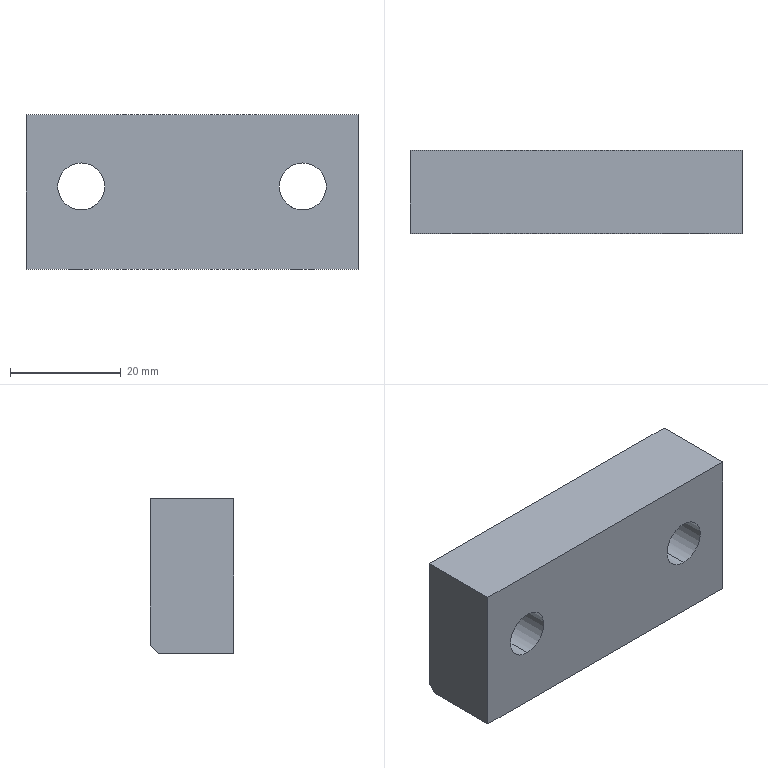Component | SolidWorks | Q1-A12-S21-Q4E.SLDASQ-5_Q1-A12-S21-Q1E-02A-1 | 1 solid | 15 faces | box 60 x 15 x 28 mm | volume 23129 mm3 | cylinder 8 | plane 7 | commonest cylinder face diameters 8.5 x4 4.2 x4 | material Q235-Steel
build123d program:
from build123d import *

# Parameters (mm, degrees)
SKETCH1_W                  = 60
SKETCH1_H                  = 28
BOSS_EXTRUDE1_DEPTH        = 15
M5X0_8_TAPPED_HOLE1_D      = 4.2
M5X0_8_TAPPED_HOLE1_DEPTH  = 12.4
M5X0_8_TAPPED_HOLE1_TIP    = 1.262
F_8_5_8_5_DIAMETER_HOLE1_D = 8.5
CHAMFER1_SIZE              = 1.5


with BuildPart() as part:
    # Sketch1 → Boss-Extrude1 (new body)
    with BuildSketch(Plane(origin=(0, 0, 0), x_dir=(1, 0, 0), z_dir=(0, 1, 0))):
        Rectangle(SKETCH1_W, SKETCH1_H)
    extrude(amount=BOSS_EXTRUDE1_DEPTH)

    # M5x0.8 Tapped Hole1
    with Locations(Plane(origin=(0, 0, -14), x_dir=(-1, 0, 0), z_dir=(0, 0, -1))):
        with Locations((20, 7.5), (-20, 7.5)):
            Hole(M5X0_8_TAPPED_HOLE1_D / 2, depth=M5X0_8_TAPPED_HOLE1_DEPTH)
            with Locations((0, 0, -(M5X0_8_TAPPED_HOLE1_DEPTH + M5X0_8_TAPPED_HOLE1_TIP / 2))):  # 118° drill point
                Cone(0, M5X0_8_TAPPED_HOLE1_D / 2, M5X0_8_TAPPED_HOLE1_TIP, mode=Mode.SUBTRACT)

    # 8.5 _8.5_ Diameter Hole1 (through all)
    with Locations(Plane(origin=(0, 15, 0), x_dir=(1, 0, 0), z_dir=(0, 1, 0))):
        with Locations((-20, -1), (20, -1)):
            Hole(F_8_5_8_5_DIAMETER_HOLE1_D / 2)

    # Chamfer1
    chamfer1_edges = [part.edges().sort_by_distance(p)[0] for p in [
        (0, 15, -14),
    ]]
    chamfer(chamfer1_edges, length=CHAMFER1_SIZE)


solid = part.part

# Placed as in the assembly
solid = solid.moved(Location((1198.5, -55, 174), (0, 0, 0)))
STEP:
#1=COLOUR_RGB('',0.7922,0.8196,0.9333);
#2=FILL_AREA_STYLE_COLOUR('',#1);
#3=FILL_AREA_STYLE('',(#2));
#4=SURFACE_STYLE_FILL_AREA(#3);
#5=SURFACE_SIDE_STYLE('',(#4));
#6=SURFACE_STYLE_USAGE(.BOTH.,#5);
#7=PRESENTATION_STYLE_ASSIGNMENT((#6));
#8=CARTESIAN_POINT('',(46.398,-2.165,6.722));
#9=VERTEX_POINT('',#8);
#10=CARTESIAN_POINT('',(46.398,-2.165,7.057));
#11=VERTEX_POINT('',#10);
#12=CARTESIAN_POINT('',(46.398,-2.165,6.89));
#13=DIRECTION('',(0.,1.,0.));
#14=DIRECTION('',(0.,0.,1.));
#15=AXIS2_PLACEMENT_3D('',#12,#13,#14);
#16=CIRCLE('',#15,0.1673);
#17=EDGE_CURVE('',#9,#11,#16,.T.);
#18=ORIENTED_EDGE('',*,*,#17,.F.);
#19=CARTESIAN_POINT('',(46.398,-1.953,6.722));
#20=VERTEX_POINT('',#19);
#21=CARTESIAN_POINT('',(46.398,-1.575,6.722));
#22=DIRECTION('',(0.,1.,0.));
#23=VECTOR('',#22,39.37);
#24=LINE('',#21,#23);
#25=EDGE_CURVE('',#9,#20,#24,.T.);
#26=ORIENTED_EDGE('',*,*,#25,.T.);
#27=CARTESIAN_POINT('',(46.315,-1.87,6.744));
#28=VERTEX_POINT('',#27);
#29=CARTESIAN_POINT('',(46.315,-1.87,6.744));
#30=CARTESIAN_POINT('',(46.315,-1.876,6.744));
#31=CARTESIAN_POINT('',(46.316,-1.881,6.744));
#32=CARTESIAN_POINT('',(46.318,-1.892,6.743));
#33=CARTESIAN_POINT('',(46.319,-1.897,6.742));
#34=CARTESIAN_POINT('',(46.326,-1.912,6.739));
#35=CARTESIAN_POINT('',(46.332,-1.921,6.736));
#36=CARTESIAN_POINT('',(46.347,-1.936,6.73));
#37=CARTESIAN_POINT('',(46.356,-1.942,6.727));
#38=CARTESIAN_POINT('',(46.371,-1.948,6.725));
#39=CARTESIAN_POINT('',(46.376,-1.95,6.724));
#40=CARTESIAN_POINT('',(46.387,-1.952,6.723));
#41=CARTESIAN_POINT('',(46.392,-1.953,6.722));
#42=CARTESIAN_POINT('',(46.398,-1.953,6.722));
#43=B_SPLINE_CURVE_WITH_KNOTS('',3,(#29,#30,#31,#32,#33,#34,#35,#36,#37,#38,#39,#40,#41,#42),.UNSPECIFIED.,.F.,.F.,(4,2,2,2,2,2,4),(0.,0.0004174,0.0008349,0.00167,0.002505,0.002922,0.003339),.UNSPECIFIED.);
#44=EDGE_CURVE('',#28,#20,#43,.T.);
#45=ORIENTED_EDGE('',*,*,#44,.F.);
#46=CARTESIAN_POINT('',(46.398,-1.787,6.722));
#47=VERTEX_POINT('',#46);
#48=CARTESIAN_POINT('',(46.398,-1.787,6.722));
#49=CARTESIAN_POINT('',(46.392,-1.787,6.722));
#50=CARTESIAN_POINT('',(46.387,-1.788,6.723));
#51=CARTESIAN_POINT('',(46.376,-1.79,6.724));
#52=CARTESIAN_POINT('',(46.371,-1.792,6.725));
#53=CARTESIAN_POINT('',(46.356,-1.798,6.727));
#54=CARTESIAN_POINT('',(46.347,-1.804,6.73));
#55=CARTESIAN_POINT('',(46.335,-1.815,6.734));
#56=CARTESIAN_POINT('',(46.332,-1.82,6.736));
#57=CARTESIAN_POINT('',(46.326,-1.828,6.738));
#58=CARTESIAN_POINT('',(46.323,-1.833,6.74));
#59=CARTESIAN_POINT('',(46.319,-1.843,6.742));
#60=CARTESIAN_POINT('',(46.318,-1.848,6.743));
#61=CARTESIAN_POINT('',(46.316,-1.859,6.744));
#62=CARTESIAN_POINT('',(46.315,-1.865,6.744));
#63=CARTESIAN_POINT('',(46.315,-1.87,6.744));
#64=B_SPLINE_CURVE_WITH_KNOTS('',3,(#48,#49,#50,#51,#52,#53,#54,#55,#56,#57,#58,#59,#60,#61,#62,#63),.UNSPECIFIED.,.F.,.F.,(4,2,2,2,2,2,2,4),(0.01001,0.01043,0.01084,0.01168,0.01209,0.01251,0.01292,0.01334),.UNSPECIFIED.);
#65=EDGE_CURVE('',#47,#28,#64,.T.);
#66=ORIENTED_EDGE('',*,*,#65,.F.);
#67=CARTESIAN_POINT('',(46.398,-1.575,6.722));
#68=VERTEX_POINT('',#67);
#69=CARTESIAN_POINT('',(46.398,-1.575,6.722));
#70=DIRECTION('',(0.,1.,0.));
#71=VECTOR('',#70,39.37);
#72=LINE('',#69,#71);
#73=EDGE_CURVE('',#47,#68,#72,.T.);
#74=ORIENTED_EDGE('',*,*,#73,.T.);
#75=CARTESIAN_POINT('',(46.398,-1.575,7.057));
#76=VERTEX_POINT('',#75);
#77=CARTESIAN_POINT('',(46.398,-1.575,6.89));
#78=DIRECTION('',(0.,1.,0.));
#79=DIRECTION('',(0.,0.,1.));
#80=AXIS2_PLACEMENT_3D('',#77,#78,#79);
#81=CIRCLE('',#80,0.1673);
#82=EDGE_CURVE('',#68,#76,#81,.T.);
#83=ORIENTED_EDGE('',*,*,#82,.T.);
#84=CARTESIAN_POINT('',(46.398,-1.575,7.057));
#85=DIRECTION('',(0.,1.,0.));
#86=VECTOR('',#85,39.37);
#87=LINE('',#84,#86);
#88=EDGE_CURVE('',#11,#76,#87,.T.);
#89=ORIENTED_EDGE('',*,*,#88,.F.);
#90=EDGE_LOOP('',(#18,#26,#45,#66,#74,#83,#89));
#91=FACE_OUTER_BOUND('',#90,.T.);
#92=CARTESIAN_POINT('',(46.398,-1.575,6.89));
#93=DIRECTION('',(0.,1.,0.));
#94=DIRECTION('',(0.,0.,1.));
#95=AXIS2_PLACEMENT_3D('',#92,#93,#94);
#96=CYLINDRICAL_SURFACE('',#95,0.1673);
#97=ADVANCED_FACE('',(#91),#96,.F.);
#98=CARTESIAN_POINT('',(47.972,-2.165,6.722));
#99=VERTEX_POINT('',#98);
#100=CARTESIAN_POINT('',(47.972,-2.165,7.057));
#101=VERTEX_POINT('',#100);
#102=CARTESIAN_POINT('',(47.972,-2.165,6.89));
#103=DIRECTION('',(0.,1.,0.));
#104=DIRECTION('',(0.,0.,1.));
#105=AXIS2_PLACEMENT_3D('',#102,#103,#104);
#106=CIRCLE('',#105,0.1673);
#107=EDGE_CURVE('',#99,#101,#106,.T.);
#108=ORIENTED_EDGE('',*,*,#107,.F.);
#109=CARTESIAN_POINT('',(47.972,-1.953,6.722));
#110=VERTEX_POINT('',#109);
#111=CARTESIAN_POINT('',(47.972,-1.575,6.722));
#112=DIRECTION('',(0.,1.,0.));
#113=VECTOR('',#112,39.37);
#114=LINE('',#111,#113);
#115=EDGE_CURVE('',#99,#110,#114,.T.);
#116=ORIENTED_EDGE('',*,*,#115,.T.);
#117=CARTESIAN_POINT('',(47.89,-1.87,6.744));
#118=VERTEX_POINT('',#117);
#119=CARTESIAN_POINT('',(47.89,-1.87,6.744));
#120=CARTESIAN_POINT('',(47.89,-1.876,6.744));
#121=CARTESIAN_POINT('',(47.89,-1.881,6.744));
#122=CARTESIAN_POINT('',(47.892,-1.892,6.743));
#123=CARTESIAN_POINT('',(47.894,-1.897,6.742));
#124=CARTESIAN_POINT('',(47.9,-1.912,6.739));
#125=CARTESIAN_POINT('',(47.906,-1.921,6.736));
#126=CARTESIAN_POINT('',(47.921,-1.936,6.73));
#127=CARTESIAN_POINT('',(47.931,-1.942,6.727));
#128=CARTESIAN_POINT('',(47.945,-1.948,6.725));
#129=CARTESIAN_POINT('',(47.951,-1.95,6.724));
#130=CARTESIAN_POINT('',(47.961,-1.952,6.723));
#131=CARTESIAN_POINT('',(47.967,-1.953,6.722));
#132=CARTESIAN_POINT('',(47.972,-1.953,6.722));
#133=B_SPLINE_CURVE_WITH_KNOTS('',3,(#119,#120,#121,#122,#123,#124,#125,#126,#127,#128,#129,#130,#131,#132),.UNSPECIFIED.,.F.,.F.,(4,2,2,2,2,2,4),(0.,0.0004174,0.0008349,0.00167,0.002505,0.002922,0.003339),.UNSPECIFIED.);
#134=EDGE_CURVE('',#118,#110,#133,.T.);
#135=ORIENTED_EDGE('',*,*,#134,.F.);
#136=CARTESIAN_POINT('',(47.972,-1.787,6.722));
#137=VERTEX_POINT('',#136);
#138=CARTESIAN_POINT('',(47.972,-1.787,6.722));
#139=CARTESIAN_POINT('',(47.967,-1.787,6.722));
#140=CARTESIAN_POINT('',(47.961,-1.788,6.723));
#141=CARTESIAN_POINT('',(47.951,-1.79,6.724));
#142=CARTESIAN_POINT('',(47.945,-1.792,6.725));
#143=CARTESIAN_POINT('',(47.93,-1.798,6.727));
#144=CARTESIAN_POINT('',(47.921,-1.804,6.73));
#145=CARTESIAN_POINT('',(47.91,-1.815,6.734));
#146=CARTESIAN_POINT('',(47.907,-1.82,6.736));
#147=CARTESIAN_POINT('',(47.901,-1.828,6.738));
#148=CARTESIAN_POINT('',(47.898,-1.833,6.74));
#149=CARTESIAN_POINT('',(47.894,-1.843,6.742));
#150=CARTESIAN_POINT('',(47.893,-1.848,6.743));
#151=CARTESIAN_POINT('',(47.89,-1.859,6.744));
#152=CARTESIAN_POINT('',(47.89,-1.865,6.744));
#153=CARTESIAN_POINT('',(47.89,-1.87,6.744));
#154=B_SPLINE_CURVE_WITH_KNOTS('',3,(#138,#139,#140,#141,#142,#143,#144,#145,#146,#147,#148,#149,#150,#151,#152,#153),.UNSPECIFIED.,.F.,.F.,(4,2,2,2,2,2,2,4),(0.01001,0.01043,0.01084,0.01168,0.01209,0.01251,0.01292,0.01334),.UNSPECIFIED.);
#155=EDGE_CURVE('',#137,#118,#154,.T.);
#156=ORIENTED_EDGE('',*,*,#155,.F.);
#157=CARTESIAN_POINT('',(47.972,-1.575,6.722));
#158=VERTEX_POINT('',#157);
#159=CARTESIAN_POINT('',(47.972,-1.575,6.722));
#160=DIRECTION('',(0.,1.,0.));
#161=VECTOR('',#160,39.37);
#162=LINE('',#159,#161);
#163=EDGE_CURVE('',#137,#158,#162,.T.);
#164=ORIENTED_EDGE('',*,*,#163,.T.);
#165=CARTESIAN_POINT('',(47.972,-1.575,7.057));
#166=VERTEX_POINT('',#165);
#167=CARTESIAN_POINT('',(47.972,-1.575,6.89));
#168=DIRECTION('',(0.,1.,0.));
#169=DIRECTION('',(0.,0.,1.));
#170=AXIS2_PLACEMENT_3D('',#167,#168,#169);
#171=CIRCLE('',#170,0.1673);
#172=EDGE_CURVE('',#158,#166,#171,.T.);
#173=ORIENTED_EDGE('',*,*,#172,.T.);
#174=CARTESIAN_POINT('',(47.972,-1.575,7.057));
#175=DIRECTION('',(0.,1.,0.));
#176=VECTOR('',#175,39.37);
#177=LINE('',#174,#176);
#178=EDGE_CURVE('',#101,#166,#177,.T.);
#179=ORIENTED_EDGE('',*,*,#178,.F.);
#180=EDGE_LOOP('',(#108,#116,#135,#156,#164,#173,#179));
#181=FACE_OUTER_BOUND('',#180,.T.);
#182=CARTESIAN_POINT('',(47.972,-1.575,6.89));
#183=DIRECTION('',(0.,1.,0.));
#184=DIRECTION('',(0.,0.,1.));
#185=AXIS2_PLACEMENT_3D('',#182,#183,#184);
#186=CYLINDRICAL_SURFACE('',#185,0.1673);
#187=ADVANCED_FACE('',(#181),#186,.F.);
#188=ORIENTED_EDGE('',*,*,#44,.T.);
#189=CARTESIAN_POINT('',(46.48,-1.87,6.744));
#190=VERTEX_POINT('',#189);
#191=CARTESIAN_POINT('',(46.398,-1.953,6.722));
#192=CARTESIAN_POINT('',(46.403,-1.953,6.722));
#193=CARTESIAN_POINT('',(46.409,-1.952,6.723));
#194=CARTESIAN_POINT('',(46.419,-1.95,6.724));
#195=CARTESIAN_POINT('',(46.425,-1.948,6.725));
#196=CARTESIAN_POINT('',(46.435,-1.944,6.727));
#197=CARTESIAN_POINT('',(46.439,-1.942,6.728));
#198=CARTESIAN_POINT('',(46.448,-1.936,6.73));
#199=CARTESIAN_POINT('',(46.452,-1.932,6.732));
#200=CARTESIAN_POINT('',(46.464,-1.921,6.736));
#201=CARTESIAN_POINT('',(46.47,-1.912,6.739));
#202=CARTESIAN_POINT('',(46.476,-1.897,6.742));
#203=CARTESIAN_POINT('',(46.478,-1.892,6.743));
#204=CARTESIAN_POINT('',(46.48,-1.881,6.744));
#205=CARTESIAN_POINT('',(46.48,-1.876,6.744));
#206=CARTESIAN_POINT('',(46.48,-1.87,6.744));
#207=B_SPLINE_CURVE_WITH_KNOTS('',3,(#191,#192,#193,#194,#195,#196,#197,#198,#199,#200,#201,#202,#203,#204,#205,#206),.UNSPECIFIED.,.F.,.F.,(4,2,2,2,2,2,2,4),(0.003339,0.003757,0.004174,0.004591,0.005008,0.005842,0.006259,0.006676),.UNSPECIFIED.);
#208=EDGE_CURVE('',#20,#190,#207,.T.);
#209=ORIENTED_EDGE('',*,*,#208,.T.);
#210=CARTESIAN_POINT('',(46.48,-1.87,6.299));
#211=VERTEX_POINT('',#210);
#212=CARTESIAN_POINT('',(46.48,-1.87,6.299));
#213=DIRECTION('',(0.,0.,-1.));
#214=VECTOR('',#213,39.37);
#215=LINE('',#212,#214);
#216=EDGE_CURVE('',#190,#211,#215,.T.);
#217=ORIENTED_EDGE('',*,*,#216,.T.);
#218=CARTESIAN_POINT('',(46.315,-1.87,6.299));
#219=VERTEX_POINT('',#218);
#220=CARTESIAN_POINT('',(46.398,-1.87,6.299));
#221=DIRECTION('',(0.,0.,-1.));
#222=DIRECTION('',(-1.,0.,0.));
#223=AXIS2_PLACEMENT_3D('',#220,#221,#222);
#224=CIRCLE('',#223,0.08268);
#225=EDGE_CURVE('',#211,#219,#224,.T.);
#226=ORIENTED_EDGE('',*,*,#225,.T.);
#227=CARTESIAN_POINT('',(46.315,-1.87,6.299));
#228=DIRECTION('',(0.,0.,-1.));
#229=VECTOR('',#228,39.37);
#230=LINE('',#227,#229);
#231=EDGE_CURVE('',#28,#219,#230,.T.);
#232=ORIENTED_EDGE('',*,*,#231,.F.);
#233=EDGE_LOOP('',(#188,#209,#217,#226,#232));
#234=FACE_OUTER_BOUND('',#233,.T.);
#235=CARTESIAN_POINT('',(46.398,-1.87,6.299));
#236=DIRECTION('',(0.,0.,-1.));
#237=DIRECTION('',(-1.,0.,0.));
#238=AXIS2_PLACEMENT_3D('',#235,#236,#237);
#239=CYLINDRICAL_SURFACE('',#238,0.08268);
#240=ADVANCED_FACE('',(#234),#239,.F.);
#241=ORIENTED_EDGE('',*,*,#134,.T.);
#242=CARTESIAN_POINT('',(48.055,-1.87,6.744));
#243=VERTEX_POINT('',#242);
#244=CARTESIAN_POINT('',(47.972,-1.953,6.722));
#245=CARTESIAN_POINT('',(47.978,-1.953,6.722));
#246=CARTESIAN_POINT('',(47.984,-1.952,6.723));
#247=CARTESIAN_POINT('',(47.994,-1.95,6.724));
#248=CARTESIAN_POINT('',(47.999,-1.948,6.725));
#249=CARTESIAN_POINT('',(48.009,-1.944,6.727));
#250=CARTESIAN_POINT('',(48.014,-1.942,6.728));
#251=CARTESIAN_POINT('',(48.023,-1.936,6.73));
#252=CARTESIAN_POINT('',(48.027,-1.932,6.732));
#253=CARTESIAN_POINT('',(48.039,-1.921,6.736));
#254=CARTESIAN_POINT('',(48.045,-1.912,6.739));
#255=CARTESIAN_POINT('',(48.051,-1.897,6.742));
#256=CARTESIAN_POINT('',(48.052,-1.892,6.743));
#257=CARTESIAN_POINT('',(48.055,-1.881,6.744));
#258=CARTESIAN_POINT('',(48.055,-1.876,6.744));
#259=CARTESIAN_POINT('',(48.055,-1.87,6.744));
#260=B_SPLINE_CURVE_WITH_KNOTS('',3,(#244,#245,#246,#247,#248,#249,#250,#251,#252,#253,#254,#255,#256,#257,#258,#259),.UNSPECIFIED.,.F.,.F.,(4,2,2,2,2,2,2,4),(0.003339,0.003757,0.004174,0.004591,0.005008,0.005842,0.006259,0.006676),.UNSPECIFIED.);
#261=EDGE_CURVE('',#110,#243,#260,.T.);
#262=ORIENTED_EDGE('',*,*,#261,.T.);
#263=CARTESIAN_POINT('',(48.055,-1.87,6.299));
#264=VERTEX_POINT('',#263);
#265=CARTESIAN_POINT('',(48.055,-1.87,6.299));
#266=DIRECTION('',(0.,0.,-1.));
#267=VECTOR('',#266,39.37);
#268=LINE('',#265,#267);
#269=EDGE_CURVE('',#243,#264,#268,.T.);
#270=ORIENTED_EDGE('',*,*,#269,.T.);
#271=CARTESIAN_POINT('',(47.89,-1.87,6.299));
#272=VERTEX_POINT('',#271);
#273=CARTESIAN_POINT('',(47.972,-1.87,6.299));
#274=DIRECTION('',(0.,0.,-1.));
#275=DIRECTION('',(-1.,0.,0.));
#276=AXIS2_PLACEMENT_3D('',#273,#274,#275);
#277=CIRCLE('',#276,0.08268);
#278=EDGE_CURVE('',#264,#272,#277,.T.);
#279=ORIENTED_EDGE('',*,*,#278,.T.);
#280=CARTESIAN_POINT('',(47.89,-1.87,6.299));
#281=DIRECTION('',(0.,0.,-1.));
#282=VECTOR('',#281,39.37);
#283=LINE('',#280,#282);
#284=EDGE_CURVE('',#118,#272,#283,.T.);
#285=ORIENTED_EDGE('',*,*,#284,.F.);
#286=EDGE_LOOP('',(#241,#262,#270,#279,#285));
#287=FACE_OUTER_BOUND('',#286,.T.);
#288=CARTESIAN_POINT('',(47.972,-1.87,6.299));
#289=DIRECTION('',(0.,0.,-1.));
#290=DIRECTION('',(-1.,0.,0.));
#291=AXIS2_PLACEMENT_3D('',#288,#289,#290);
#292=CYLINDRICAL_SURFACE('',#291,0.08268);
#293=ADVANCED_FACE('',(#287),#292,.F.);
#294=CARTESIAN_POINT('',(48.366,-1.634,6.299));
#295=VERTEX_POINT('',#294);
#296=CARTESIAN_POINT('',(48.366,-2.165,6.299));
#297=VERTEX_POINT('',#296);
#298=CARTESIAN_POINT('',(48.366,-1.575,6.299));
#299=DIRECTION('',(0.,-1.,0.));
#300=VECTOR('',#299,39.37);
#301=LINE('',#298,#300);
#302=EDGE_CURVE('',#295,#297,#301,.T.);
#303=ORIENTED_EDGE('',*,*,#302,.F.);
#304=CARTESIAN_POINT('',(48.366,-1.575,6.358));
#305=VERTEX_POINT('',#304);
#306=CARTESIAN_POINT('',(48.366,-1.575,6.358));
#307=DIRECTION('',(0.,0.7071,0.7071));
#308=VECTOR('',#307,39.37);
#309=LINE('',#306,#308);
#310=EDGE_CURVE('',#295,#305,#309,.T.);
#311=ORIENTED_EDGE('',*,*,#310,.T.);
#312=CARTESIAN_POINT('',(48.366,-1.575,7.402));
#313=VERTEX_POINT('',#312);
#314=CARTESIAN_POINT('',(48.366,-1.575,7.402));
#315=DIRECTION('',(0.,0.,-1.));
#316=VECTOR('',#315,39.37);
#317=LINE('',#314,#316);
#318=EDGE_CURVE('',#313,#305,#317,.T.);
#319=ORIENTED_EDGE('',*,*,#318,.F.);
#320=CARTESIAN_POINT('',(48.366,-2.165,7.402));
#321=VERTEX_POINT('',#320);
#322=CARTESIAN_POINT('',(48.366,-1.575,7.402));
#323=DIRECTION('',(0.,-1.,0.));
#324=VECTOR('',#323,39.37);
#325=LINE('',#322,#324);
#326=EDGE_CURVE('',#313,#321,#325,.T.);
#327=ORIENTED_EDGE('',*,*,#326,.T.);
#328=CARTESIAN_POINT('',(48.366,-2.165,7.402));
#329=DIRECTION('',(0.,0.,-1.));
#330=VECTOR('',#329,39.37);
#331=LINE('',#328,#330);
#332=EDGE_CURVE('',#321,#297,#331,.T.);
#333=ORIENTED_EDGE('',*,*,#332,.T.);
#334=EDGE_LOOP('',(#303,#311,#319,#327,#333));
#335=FACE_OUTER_BOUND('',#334,.T.);
#336=CARTESIAN_POINT('',(48.366,-1.575,7.402));
#337=DIRECTION('',(-1.,0.,0.));
#338=DIRECTION('',(0.,0.,1.));
#339=AXIS2_PLACEMENT_3D('',#336,#337,#338);
#340=PLANE('',#339);
#341=ADVANCED_FACE('',(#335),#340,.F.);
#342=CARTESIAN_POINT('',(46.398,-1.87,6.299));
#343=DIRECTION('',(0.,0.,-1.));
#344=DIRECTION('',(-1.,0.,0.));
#345=AXIS2_PLACEMENT_3D('',#342,#343,#344);
#346=CIRCLE('',#345,0.08268);
#347=EDGE_CURVE('',#219,#211,#346,.T.);
#348=ORIENTED_EDGE('',*,*,#347,.F.);
#349=ORIENTED_EDGE('',*,*,#225,.F.);
#350=EDGE_LOOP('',(#348,#349));
#351=FACE_BOUND('',#350,.T.);
#352=CARTESIAN_POINT('',(47.972,-1.87,6.299));
#353=DIRECTION('',(0.,0.,-1.));
#354=DIRECTION('',(-1.,0.,0.));
#355=AXIS2_PLACEMENT_3D('',#352,#353,#354);
#356=CIRCLE('',#355,0.08268);
#357=EDGE_CURVE('',#272,#264,#356,.T.);
#358=ORIENTED_EDGE('',*,*,#357,.F.);
#359=ORIENTED_EDGE('',*,*,#278,.F.);
#360=EDGE_LOOP('',(#358,#359));
#361=FACE_BOUND('',#360,.T.);
#362=CARTESIAN_POINT('',(46.004,-1.634,6.299));
#363=VERTEX_POINT('',#362);
#364=CARTESIAN_POINT('',(46.004,-2.165,6.299));
#365=VERTEX_POINT('',#364);
#366=CARTESIAN_POINT('',(46.004,-1.575,6.299));
#367=DIRECTION('',(0.,-1.,0.));
#368=VECTOR('',#367,39.37);
#369=LINE('',#366,#368);
#370=EDGE_CURVE('',#363,#365,#369,.T.);
#371=ORIENTED_EDGE('',*,*,#370,.F.);
#372=CARTESIAN_POINT('',(46.004,-1.634,6.299));
#373=DIRECTION('',(1.,0.,0.));
#374=VECTOR('',#373,39.37);
#375=LINE('',#372,#374);
#376=EDGE_CURVE('',#363,#295,#375,.T.);
#377=ORIENTED_EDGE('',*,*,#376,.T.);
#378=ORIENTED_EDGE('',*,*,#302,.T.);
#379=CARTESIAN_POINT('',(46.004,-2.165,6.299));
#380=DIRECTION('',(-1.,0.,0.));
#381=VECTOR('',#380,39.37);
#382=LINE('',#379,#381);
#383=EDGE_CURVE('',#297,#365,#382,.T.);
#384=ORIENTED_EDGE('',*,*,#383,.T.);
#385=EDGE_LOOP('',(#371,#377,#378,#384));
#386=FACE_OUTER_BOUND('',#385,.T.);
#387=CARTESIAN_POINT('',(46.004,-1.575,6.299));
#388=DIRECTION('',(0.,0.,1.));
#389=DIRECTION('',(1.,0.,0.));
#390=AXIS2_PLACEMENT_3D('',#387,#388,#389);
#391=PLANE('',#390);
#392=ADVANCED_FACE('',(#351,#361,#386),#391,.F.);
#393=CARTESIAN_POINT('',(46.004,-1.575,6.358));
#394=VERTEX_POINT('',#393);
#395=CARTESIAN_POINT('',(46.004,-1.575,7.402));
#396=VERTEX_POINT('',#395);
#397=CARTESIAN_POINT('',(46.004,-1.575,7.402));
#398=DIRECTION('',(0.,0.,1.));
#399=VECTOR('',#398,39.37);
#400=LINE('',#397,#399);
#401=EDGE_CURVE('',#394,#396,#400,.T.);
#402=ORIENTED_EDGE('',*,*,#401,.F.);
#403=CARTESIAN_POINT('',(46.004,-1.575,6.358));
#404=DIRECTION('',(0.,-0.7071,-0.7071));
#405=VECTOR('',#404,39.37);
#406=LINE('',#403,#405);
#407=EDGE_CURVE('',#394,#363,#406,.T.);
#408=ORIENTED_EDGE('',*,*,#407,.T.);
#409=ORIENTED_EDGE('',*,*,#370,.T.);
#410=CARTESIAN_POINT('',(46.004,-2.165,7.402));
#411=VERTEX_POINT('',#410);
#412=CARTESIAN_POINT('',(46.004,-2.165,7.402));
#413=DIRECTION('',(0.,0.,1.));
#414=VECTOR('',#413,39.37);
#415=LINE('',#412,#414);
#416=EDGE_CURVE('',#365,#411,#415,.T.);
#417=ORIENTED_EDGE('',*,*,#416,.T.);
#418=CARTESIAN_POINT('',(46.004,-1.575,7.402));
#419=DIRECTION('',(0.,-1.,0.));
#420=VECTOR('',#419,39.37);
#421=LINE('',#418,#420);
#422=EDGE_CURVE('',#396,#411,#421,.T.);
#423=ORIENTED_EDGE('',*,*,#422,.F.);
#424=EDGE_LOOP('',(#402,#408,#409,#417,#423));
#425=FACE_OUTER_BOUND('',#424,.T.);
#426=CARTESIAN_POINT('',(46.004,-1.575,7.402));
#427=DIRECTION('',(1.,0.,0.));
#428=DIRECTION('',(0.,0.,-1.));
#429=AXIS2_PLACEMENT_3D('',#426,#427,#428);
#430=PLANE('',#429);
#431=ADVANCED_FACE('',(#425),#430,.F.);
#432=CARTESIAN_POINT('',(46.004,-2.165,7.402));
#433=DIRECTION('',(1.,0.,0.));
#434=VECTOR('',#433,39.37);
#435=LINE('',#432,#434);
#436=EDGE_CURVE('',#411,#321,#435,.T.);
#437=ORIENTED_EDGE('',*,*,#436,.T.);
#438=ORIENTED_EDGE('',*,*,#326,.F.);
#439=CARTESIAN_POINT('',(46.004,-1.575,7.402));
#440=DIRECTION('',(1.,0.,0.));
#441=VECTOR('',#440,39.37);
#442=LINE('',#439,#441);
#443=EDGE_CURVE('',#396,#313,#442,.T.);
#444=ORIENTED_EDGE('',*,*,#443,.F.);
#445=ORIENTED_EDGE('',*,*,#422,.T.);
#446=EDGE_LOOP('',(#437,#438,#444,#445));
#447=FACE_OUTER_BOUND('',#446,.T.);
#448=CARTESIAN_POINT('',(46.004,-1.575,7.402));
#449=DIRECTION('',(0.,0.,-1.));
#450=DIRECTION('',(-1.,0.,0.));
#451=AXIS2_PLACEMENT_3D('',#448,#449,#450);
#452=PLANE('',#451);
#453=ADVANCED_FACE('',(#447),#452,.F.);
#454=CARTESIAN_POINT('',(46.398,-1.575,6.89));
#455=DIRECTION('',(0.,1.,0.));
#456=DIRECTION('',(0.,0.,1.));
#457=AXIS2_PLACEMENT_3D('',#454,#455,#456);
#458=CIRCLE('',#457,0.1673);
#459=EDGE_CURVE('',#76,#68,#458,.T.);
#460=ORIENTED_EDGE('',*,*,#459,.F.);
#461=ORIENTED_EDGE('',*,*,#82,.F.);
#462=EDGE_LOOP('',(#460,#461));
#463=FACE_BOUND('',#462,.T.);
#464=CARTESIAN_POINT('',(47.972,-1.575,6.89));
#465=DIRECTION('',(0.,1.,0.));
#466=DIRECTION('',(0.,0.,1.));
#467=AXIS2_PLACEMENT_3D('',#464,#465,#466);
#468=CIRCLE('',#467,0.1673);
#469=EDGE_CURVE('',#166,#158,#468,.T.);
#470=ORIENTED_EDGE('',*,*,#469,.F.);
#471=ORIENTED_EDGE('',*,*,#172,.F.);
#472=EDGE_LOOP('',(#470,#471));
#473=FACE_BOUND('',#472,.T.);
#474=ORIENTED_EDGE('',*,*,#318,.T.);
#475=CARTESIAN_POINT('',(47.185,-1.575,6.358));
#476=DIRECTION('',(-1.,0.,0.));
#477=VECTOR('',#476,39.37);
#478=LINE('',#475,#477);
#479=EDGE_CURVE('',#305,#394,#478,.T.);
#480=ORIENTED_EDGE('',*,*,#479,.T.);
#481=ORIENTED_EDGE('',*,*,#401,.T.);
#482=ORIENTED_EDGE('',*,*,#443,.T.);
#483=EDGE_LOOP('',(#474,#480,#481,#482));
#484=FACE_OUTER_BOUND('',#483,.T.);
#485=CARTESIAN_POINT('',(47.185,-1.575,6.85));
#486=DIRECTION('',(0.,-1.,0.));
#487=DIRECTION('',(0.,0.,-1.));
#488=AXIS2_PLACEMENT_3D('',#485,#486,#487);
#489=PLANE('',#488);
#490=ADVANCED_FACE('',(#463,#473,#484),#489,.F.);
#491=CARTESIAN_POINT('',(46.398,-2.165,6.89));
#492=DIRECTION('',(0.,1.,0.));
#493=DIRECTION('',(0.,0.,1.));
#494=AXIS2_PLACEMENT_3D('',#491,#492,#493);
#495=CIRCLE('',#494,0.1673);
#496=EDGE_CURVE('',#11,#9,#495,.T.);
#497=ORIENTED_EDGE('',*,*,#496,.T.);
#498=ORIENTED_EDGE('',*,*,#17,.T.);
#499=EDGE_LOOP('',(#497,#498));
#500=FACE_BOUND('',#499,.T.);
#501=CARTESIAN_POINT('',(47.972,-2.165,6.89));
#502=DIRECTION('',(0.,1.,0.));
#503=DIRECTION('',(0.,0.,1.));
#504=AXIS2_PLACEMENT_3D('',#501,#502,#503);
#505=CIRCLE('',#504,0.1673);
#506=EDGE_CURVE('',#101,#99,#505,.T.);
#507=ORIENTED_EDGE('',*,*,#506,.T.);
#508=ORIENTED_EDGE('',*,*,#107,.T.);
#509=EDGE_LOOP('',(#507,#508));
#510=FACE_BOUND('',#509,.T.);
#511=ORIENTED_EDGE('',*,*,#332,.F.);
#512=ORIENTED_EDGE('',*,*,#436,.F.);
#513=ORIENTED_EDGE('',*,*,#416,.F.);
#514=ORIENTED_EDGE('',*,*,#383,.F.);
#515=EDGE_LOOP('',(#511,#512,#513,#514));
#516=FACE_OUTER_BOUND('',#515,.T.);
#517=CARTESIAN_POINT('',(47.185,-2.165,6.85));
#518=DIRECTION('',(0.,-1.,0.));
#519=DIRECTION('',(0.,0.,-1.));
#520=AXIS2_PLACEMENT_3D('',#517,#518,#519);
#521=PLANE('',#520);
#522=ADVANCED_FACE('',(#500,#510,#516),#521,.T.);
#523=ORIENTED_EDGE('',*,*,#269,.F.);
#524=CARTESIAN_POINT('',(48.055,-1.87,6.744));
#525=CARTESIAN_POINT('',(48.055,-1.865,6.744));
#526=CARTESIAN_POINT('',(48.055,-1.859,6.744));
#527=CARTESIAN_POINT('',(48.052,-1.848,6.743));
#528=CARTESIAN_POINT('',(48.051,-1.843,6.742));
#529=CARTESIAN_POINT('',(48.047,-1.833,6.74));
#530=CARTESIAN_POINT('',(48.044,-1.828,6.738));
#531=CARTESIAN_POINT('',(48.038,-1.82,6.736));
#532=CARTESIAN_POINT('',(48.035,-1.815,6.734));
#533=CARTESIAN_POINT('',(48.027,-1.808,6.732));
#534=CARTESIAN_POINT('',(48.023,-1.804,6.73));
#535=CARTESIAN_POINT('',(48.014,-1.798,6.728));
#536=CARTESIAN_POINT('',(48.009,-1.796,6.726));
#537=CARTESIAN_POINT('',(47.999,-1.792,6.725));
#538=CARTESIAN_POINT('',(47.994,-1.79,6.724));
#539=CARTESIAN_POINT('',(47.983,-1.788,6.723));
#540=CARTESIAN_POINT('',(47.978,-1.787,6.722));
#541=CARTESIAN_POINT('',(47.972,-1.787,6.722));
#542=B_SPLINE_CURVE_WITH_KNOTS('',3,(#524,#525,#526,#527,#528,#529,#530,#531,#532,#533,#534,#535,#536,#537,#538,#539,#540,#541),.UNSPECIFIED.,.F.,.F.,(4,2,2,2,2,2,2,2,4),(0.006676,0.007093,0.00751,0.007927,0.008343,0.00876,0.009177,0.009594,0.01001),.UNSPECIFIED.);
#543=EDGE_CURVE('',#243,#137,#542,.T.);
#544=ORIENTED_EDGE('',*,*,#543,.T.);
#545=ORIENTED_EDGE('',*,*,#155,.T.);
#546=ORIENTED_EDGE('',*,*,#284,.T.);
#547=ORIENTED_EDGE('',*,*,#357,.T.);
#548=EDGE_LOOP('',(#523,#544,#545,#546,#547));
#549=FACE_OUTER_BOUND('',#548,.T.);
#550=CARTESIAN_POINT('',(47.972,-1.87,6.299));
#551=DIRECTION('',(0.,0.,-1.));
#552=DIRECTION('',(-1.,0.,0.));
#553=AXIS2_PLACEMENT_3D('',#550,#551,#552);
#554=CYLINDRICAL_SURFACE('',#553,0.08268);
#555=ADVANCED_FACE('',(#549),#554,.F.);
#556=ORIENTED_EDGE('',*,*,#216,.F.);
#557=CARTESIAN_POINT('',(46.48,-1.87,6.744));
#558=CARTESIAN_POINT('',(46.48,-1.865,6.744));
#559=CARTESIAN_POINT('',(46.48,-1.859,6.744));
#560=CARTESIAN_POINT('',(46.478,-1.848,6.743));
#561=CARTESIAN_POINT('',(46.476,-1.843,6.742));
#562=CARTESIAN_POINT('',(46.472,-1.833,6.74));
#563=CARTESIAN_POINT('',(46.469,-1.828,6.738));
#564=CARTESIAN_POINT('',(46.463,-1.82,6.736));
#565=CARTESIAN_POINT('',(46.46,-1.815,6.734));
#566=CARTESIAN_POINT('',(46.452,-1.808,6.732));
#567=CARTESIAN_POINT('',(46.448,-1.804,6.73));
#568=CARTESIAN_POINT('',(46.439,-1.798,6.728));
#569=CARTESIAN_POINT('',(46.435,-1.796,6.726));
#570=CARTESIAN_POINT('',(46.425,-1.792,6.725));
#571=CARTESIAN_POINT('',(46.419,-1.79,6.724));
#572=CARTESIAN_POINT('',(46.409,-1.788,6.723));
#573=CARTESIAN_POINT('',(46.403,-1.787,6.722));
#574=CARTESIAN_POINT('',(46.398,-1.787,6.722));
#575=B_SPLINE_CURVE_WITH_KNOTS('',3,(#557,#558,#559,#560,#561,#562,#563,#564,#565,#566,#567,#568,#569,#570,#571,#572,#573,#574),.UNSPECIFIED.,.F.,.F.,(4,2,2,2,2,2,2,2,4),(0.006676,0.007093,0.00751,0.007927,0.008343,0.00876,0.009177,0.009594,0.01001),.UNSPECIFIED.);
#576=EDGE_CURVE('',#190,#47,#575,.T.);
#577=ORIENTED_EDGE('',*,*,#576,.T.);
#578=ORIENTED_EDGE('',*,*,#65,.T.);
#579=ORIENTED_EDGE('',*,*,#231,.T.);
#580=ORIENTED_EDGE('',*,*,#347,.T.);
#581=EDGE_LOOP('',(#556,#577,#578,#579,#580));
#582=FACE_OUTER_BOUND('',#581,.T.);
#583=CARTESIAN_POINT('',(46.398,-1.87,6.299));
#584=DIRECTION('',(0.,0.,-1.));
#585=DIRECTION('',(-1.,0.,0.));
#586=AXIS2_PLACEMENT_3D('',#583,#584,#585);
#587=CYLINDRICAL_SURFACE('',#586,0.08268);
#588=ADVANCED_FACE('',(#582),#587,.F.);
#589=ORIENTED_EDGE('',*,*,#115,.F.);
#590=ORIENTED_EDGE('',*,*,#506,.F.);
#591=ORIENTED_EDGE('',*,*,#178,.T.);
#592=ORIENTED_EDGE('',*,*,#469,.T.);
#593=ORIENTED_EDGE('',*,*,#163,.F.);
#594=ORIENTED_EDGE('',*,*,#543,.F.);
#595=ORIENTED_EDGE('',*,*,#261,.F.);
#596=EDGE_LOOP('',(#589,#590,#591,#592,#593,#594,#595));
#597=FACE_OUTER_BOUND('',#596,.T.);
#598=CARTESIAN_POINT('',(47.972,-1.575,6.89));
#599=DIRECTION('',(0.,1.,0.));
#600=DIRECTION('',(0.,0.,1.));
#601=AXIS2_PLACEMENT_3D('',#598,#599,#600);
#602=CYLINDRICAL_SURFACE('',#601,0.1673);
#603=ADVANCED_FACE('',(#597),#602,.F.);
#604=ORIENTED_EDGE('',*,*,#25,.F.);
#605=ORIENTED_EDGE('',*,*,#496,.F.);
#606=ORIENTED_EDGE('',*,*,#88,.T.);
#607=ORIENTED_EDGE('',*,*,#459,.T.);
#608=ORIENTED_EDGE('',*,*,#73,.F.);
#609=ORIENTED_EDGE('',*,*,#576,.F.);
#610=ORIENTED_EDGE('',*,*,#208,.F.);
#611=EDGE_LOOP('',(#604,#605,#606,#607,#608,#609,#610));
#612=FACE_OUTER_BOUND('',#611,.T.);
#613=CARTESIAN_POINT('',(46.398,-1.575,6.89));
#614=DIRECTION('',(0.,1.,0.));
#615=DIRECTION('',(0.,0.,1.));
#616=AXIS2_PLACEMENT_3D('',#613,#614,#615);
#617=CYLINDRICAL_SURFACE('',#616,0.1673);
#618=ADVANCED_FACE('',(#612),#617,.F.);
#619=ORIENTED_EDGE('',*,*,#310,.F.);
#620=ORIENTED_EDGE('',*,*,#376,.F.);
#621=ORIENTED_EDGE('',*,*,#407,.F.);
#622=ORIENTED_EDGE('',*,*,#479,.F.);
#623=EDGE_LOOP('',(#619,#620,#621,#622));
#624=FACE_OUTER_BOUND('',#623,.T.);
#625=CARTESIAN_POINT('',(47.185,-1.575,6.358));
#626=DIRECTION('',(0.,-0.7071,0.7071));
#627=DIRECTION('',(-1.,0.,0.));
#628=AXIS2_PLACEMENT_3D('',#625,#626,#627);
#629=PLANE('',#628);
#630=ADVANCED_FACE('',(#624),#629,.F.);
#631=CLOSED_SHELL('',(#97,#187,#240,#293,#341,#392,#431,#453,#490,#522,#555,#588,#603,#618,#630));
#632=MANIFOLD_SOLID_BREP('',#631);
#633=STYLED_ITEM('',(#7),#632);
#634=PRESENTATION_LAYER_ASSIGNMENT('','',(#633));
#635=(LENGTH_UNIT()NAMED_UNIT(*)SI_UNIT($,.METRE.));
#636=LENGTH_MEASURE_WITH_UNIT(LENGTH_MEASURE(0.0254),#635);
#637=DIMENSIONAL_EXPONENTS(1.,0.,0.,0.,0.,0.,0.);
#638=(CONVERSION_BASED_UNIT('',#636)LENGTH_UNIT()NAMED_UNIT(#637));
#639=UNCERTAINTY_MEASURE_WITH_UNIT(LENGTH_MEASURE(0.00001),#638,'','');
#640=(NAMED_UNIT(*)PLANE_ANGLE_UNIT()SI_UNIT($,.RADIAN.));
#641=(NAMED_UNIT(*)SI_UNIT($,.STERADIAN.)SOLID_ANGLE_UNIT());
#642=(GEOMETRIC_REPRESENTATION_CONTEXT(3)GLOBAL_UNCERTAINTY_ASSIGNED_CONTEXT((#639))GLOBAL_UNIT_ASSIGNED_CONTEXT((#638,#640,#641))REPRESENTATION_CONTEXT('',''));
#643=MECHANICAL_DESIGN_GEOMETRIC_PRESENTATION_REPRESENTATION('',(#633),#642);
#644=CARTESIAN_POINT('',(0.,0.,0.));
#645=DIRECTION('',(0.,0.,1.));
#646=DIRECTION('',(1.,0.,0.));
#647=AXIS2_PLACEMENT_3D('',#644,#645,#646);
#648=(LENGTH_UNIT()NAMED_UNIT(*)SI_UNIT($,.METRE.));
#649=LENGTH_MEASURE_WITH_UNIT(LENGTH_MEASURE(0.0254),#648);
#650=DIMENSIONAL_EXPONENTS(1.,0.,0.,0.,0.,0.,0.);
#651=(CONVERSION_BASED_UNIT('',#649)LENGTH_UNIT()NAMED_UNIT(#650));
#652=UNCERTAINTY_MEASURE_WITH_UNIT(LENGTH_MEASURE(0.00001),#651,'','');
#653=(NAMED_UNIT(*)PLANE_ANGLE_UNIT()SI_UNIT($,.RADIAN.));
#654=(NAMED_UNIT(*)SI_UNIT($,.STERADIAN.)SOLID_ANGLE_UNIT());
#655=(GEOMETRIC_REPRESENTATION_CONTEXT(3)GLOBAL_UNCERTAINTY_ASSIGNED_CONTEXT((#652))GLOBAL_UNIT_ASSIGNED_CONTEXT((#651,#653,#654))REPRESENTATION_CONTEXT('',''));
#656=ADVANCED_BREP_SHAPE_REPRESENTATION('',(#632,#647),#655);